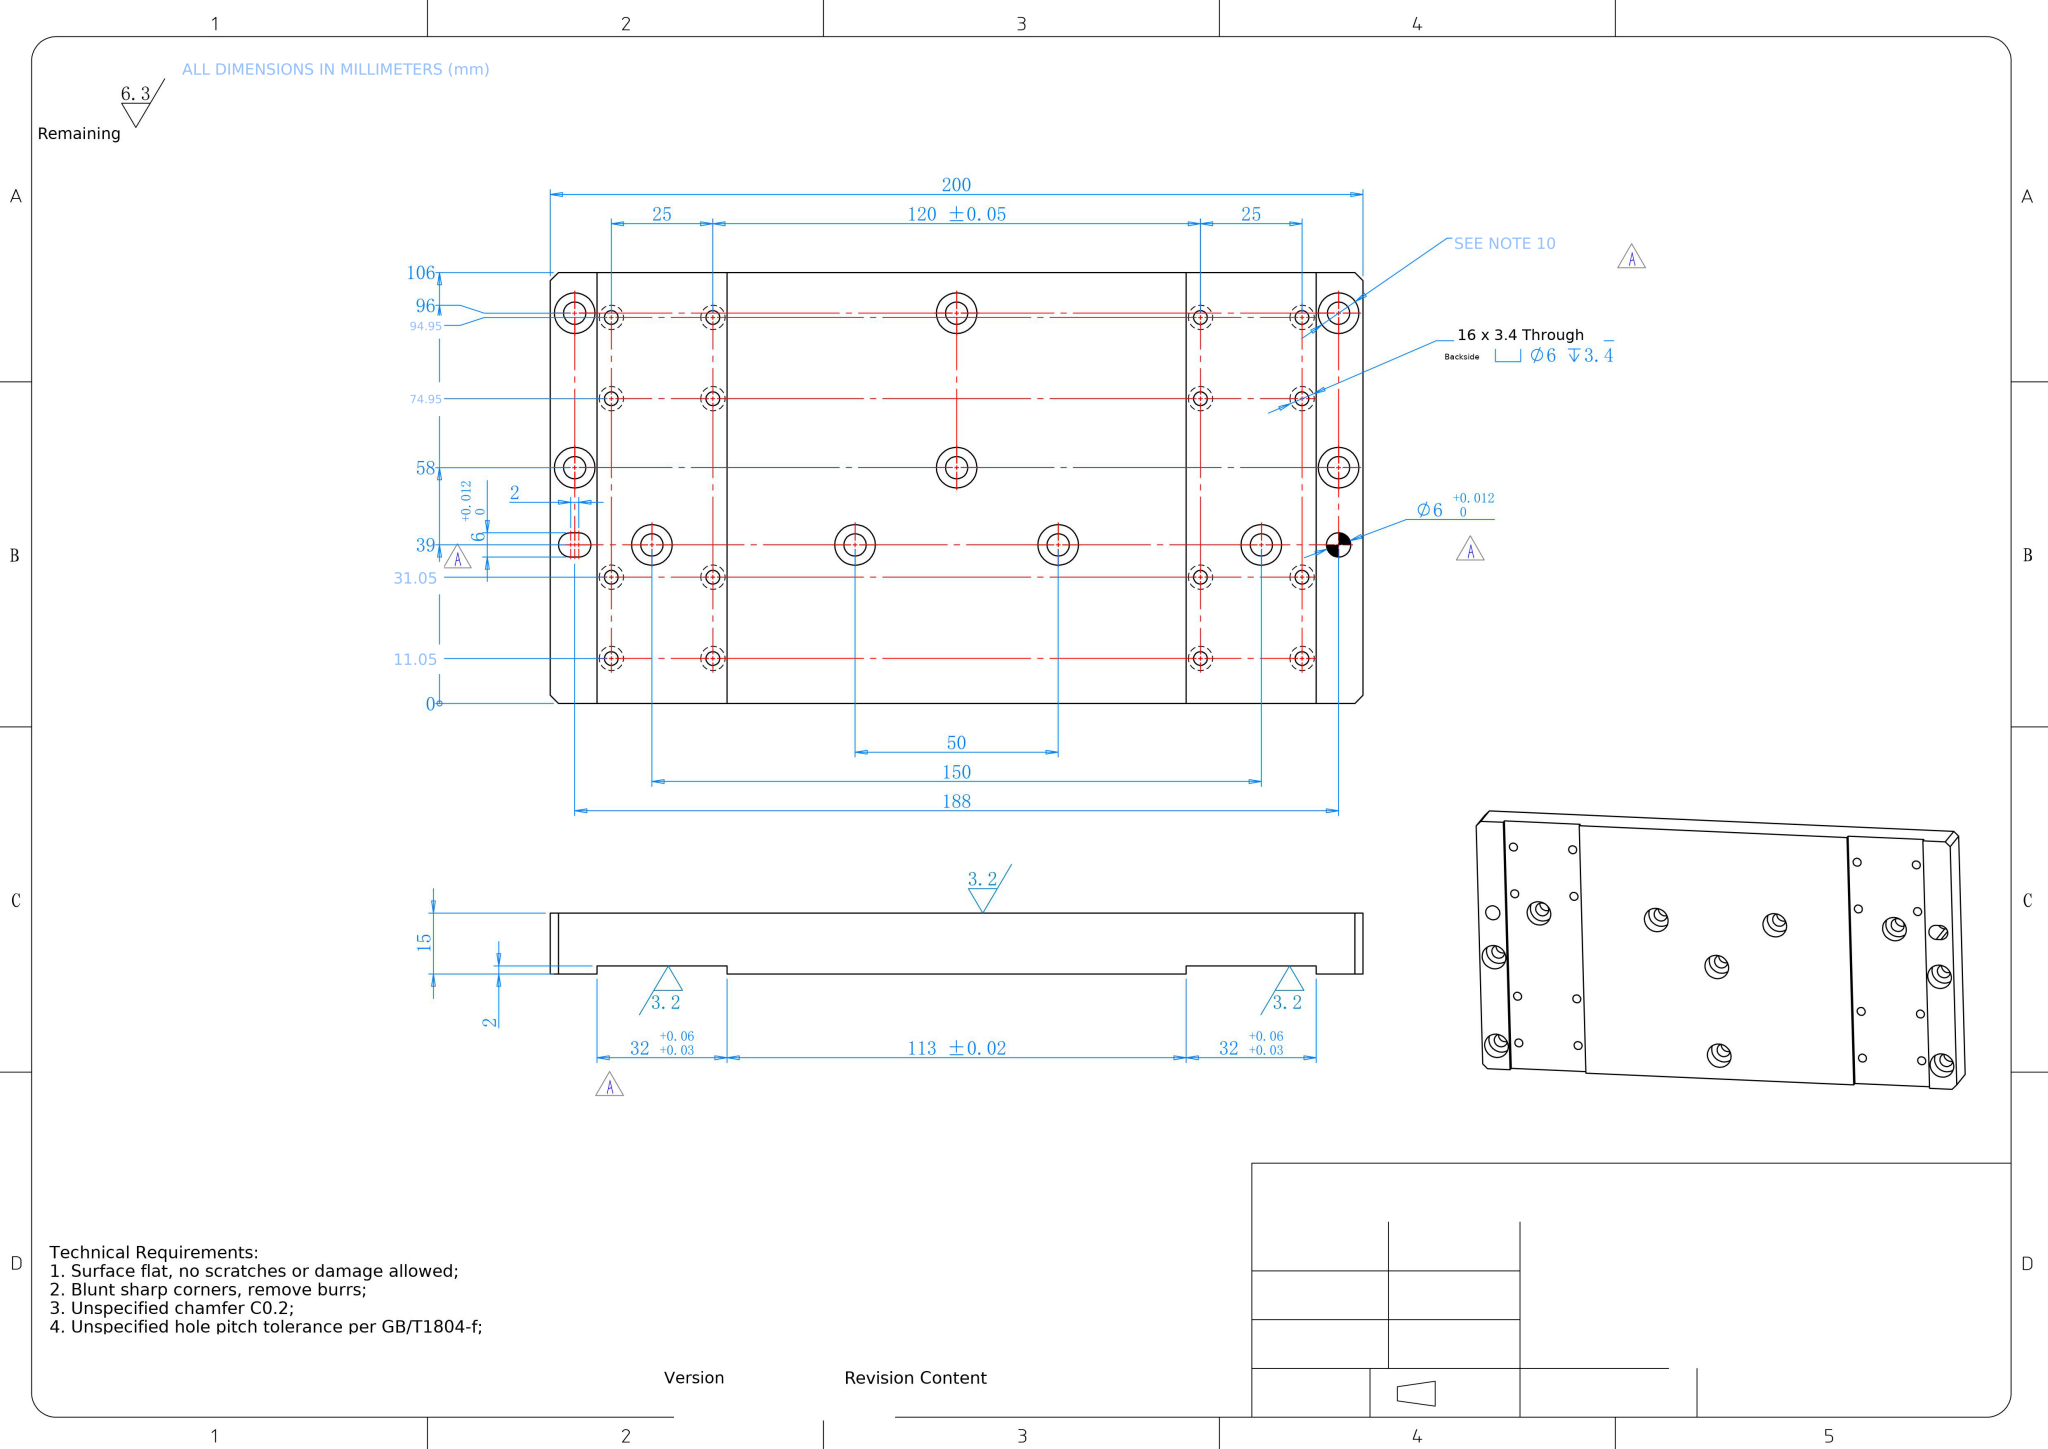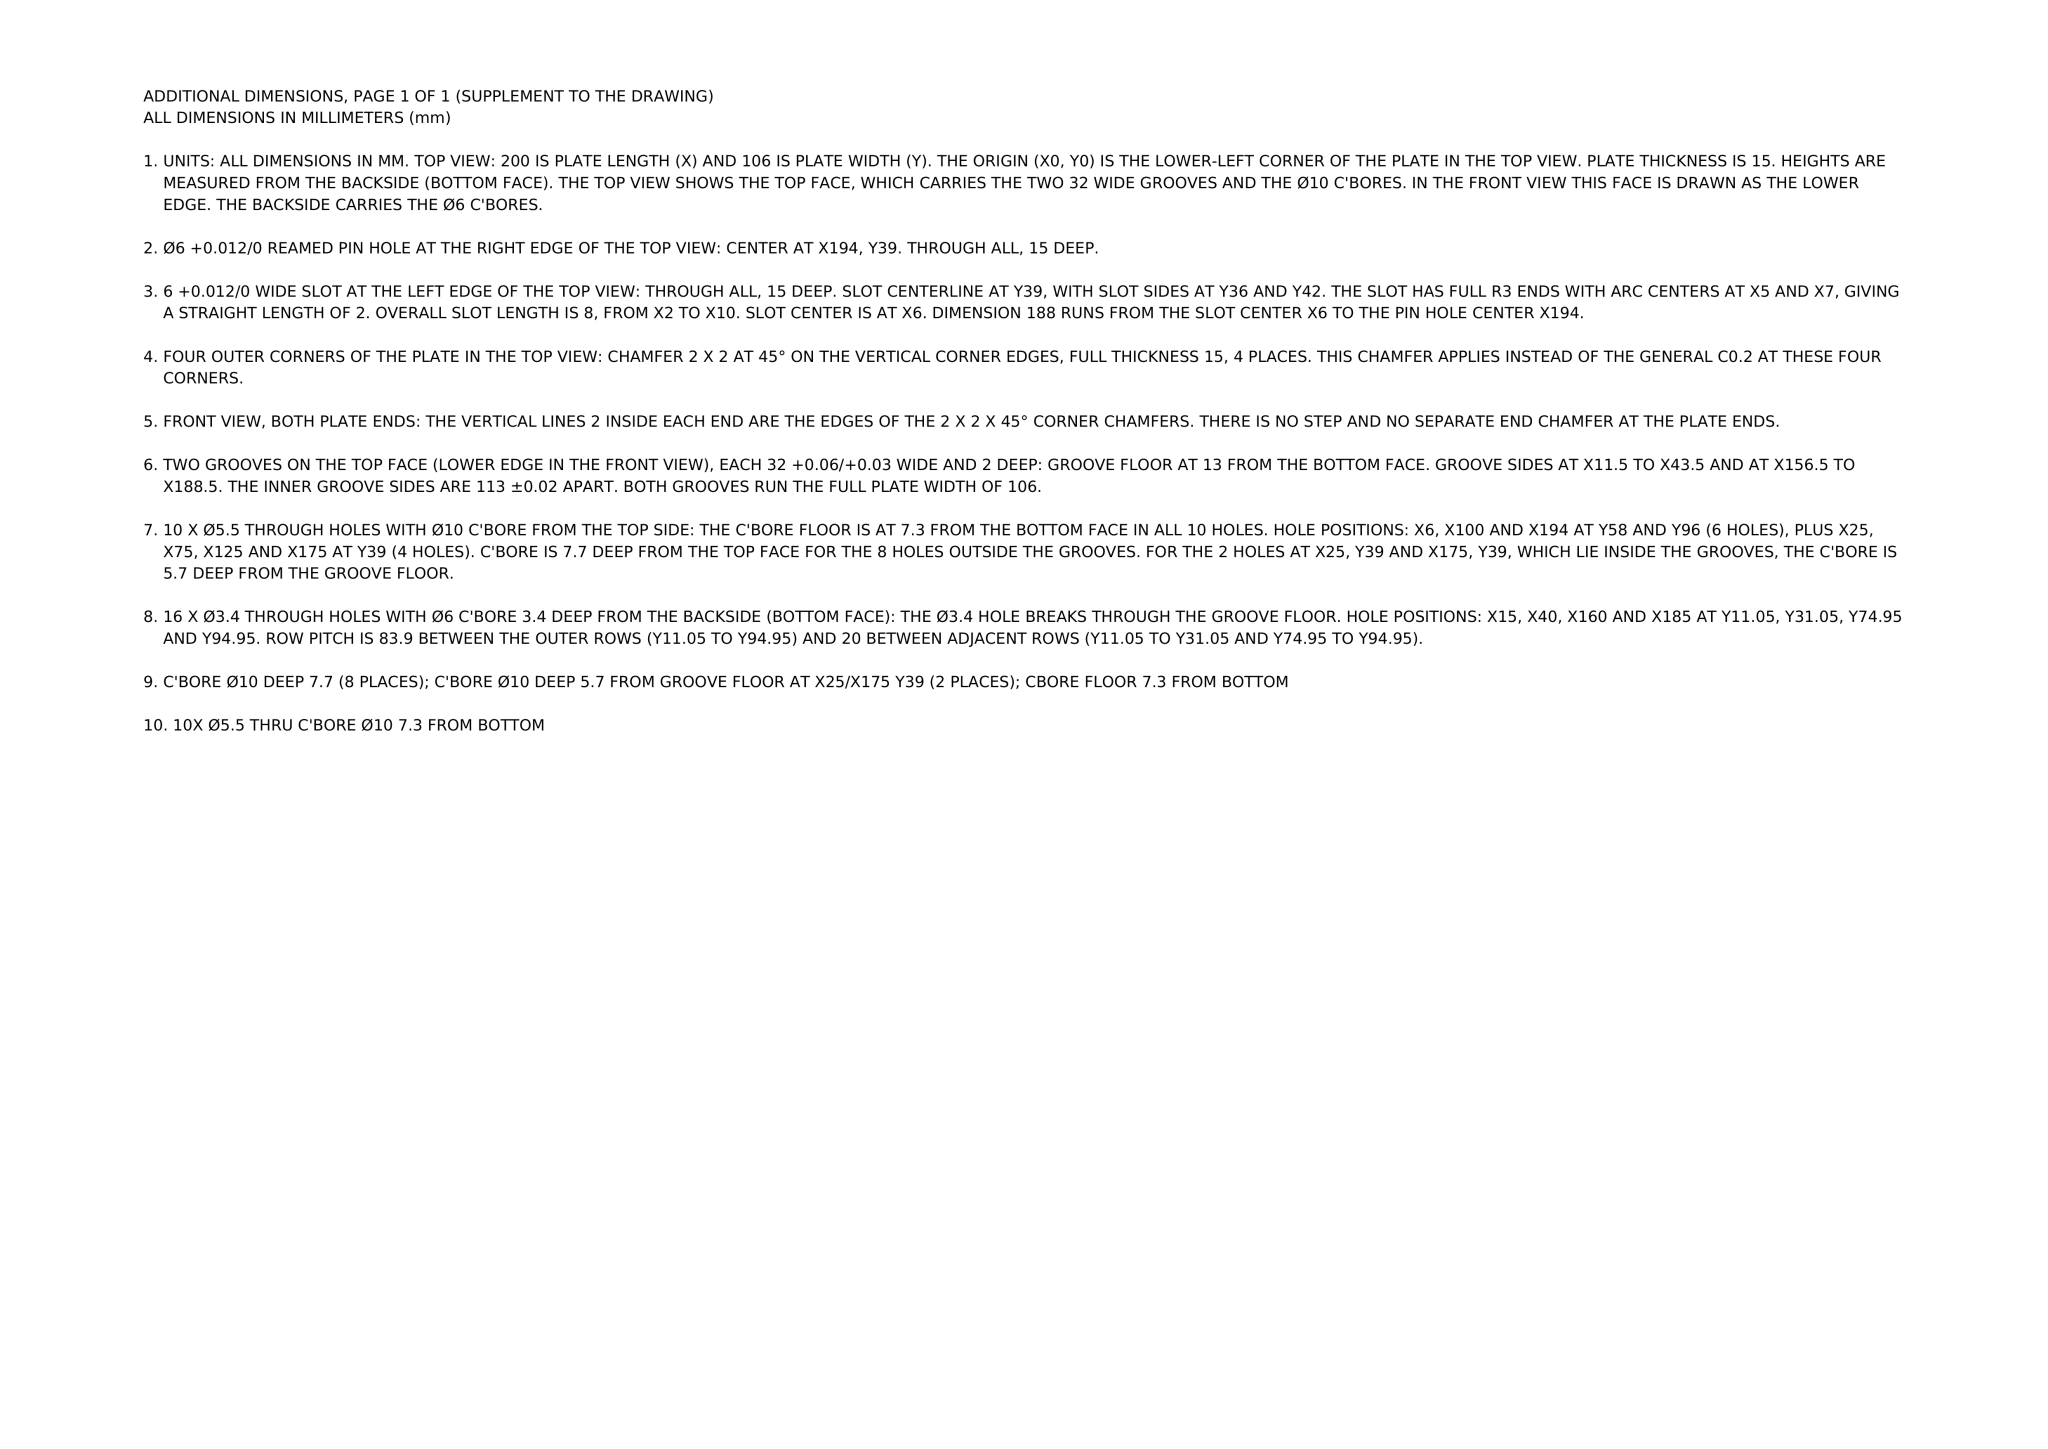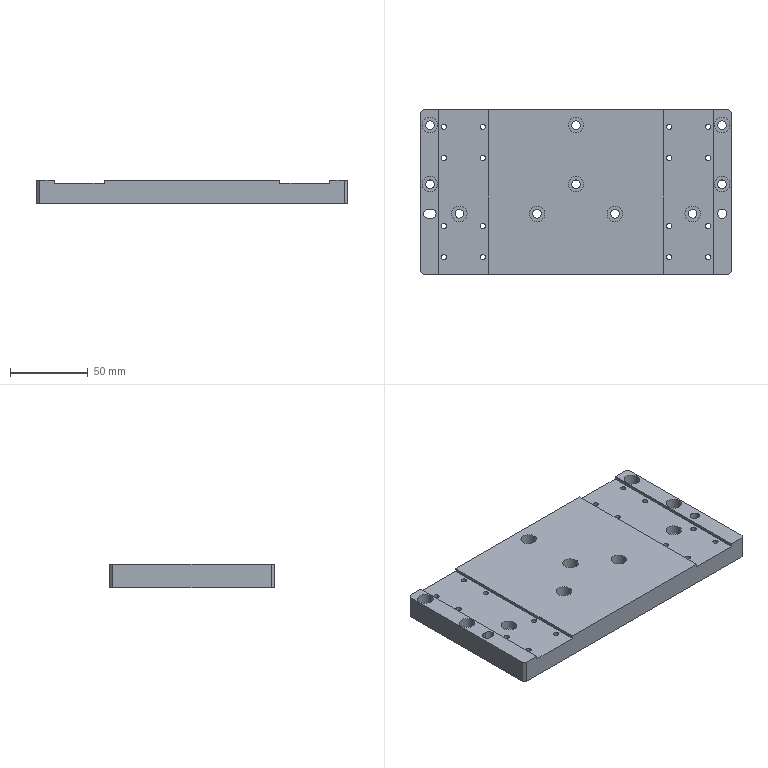Part | NX | mm | 1 solid | 155 faces | box 200 x 106 x 15 mm | volume 292883 mm3 | cylinder 109 | plane 46 | commonest cylinder face diameters 6 x37 3.4 x32 10 x20 5.5 x20